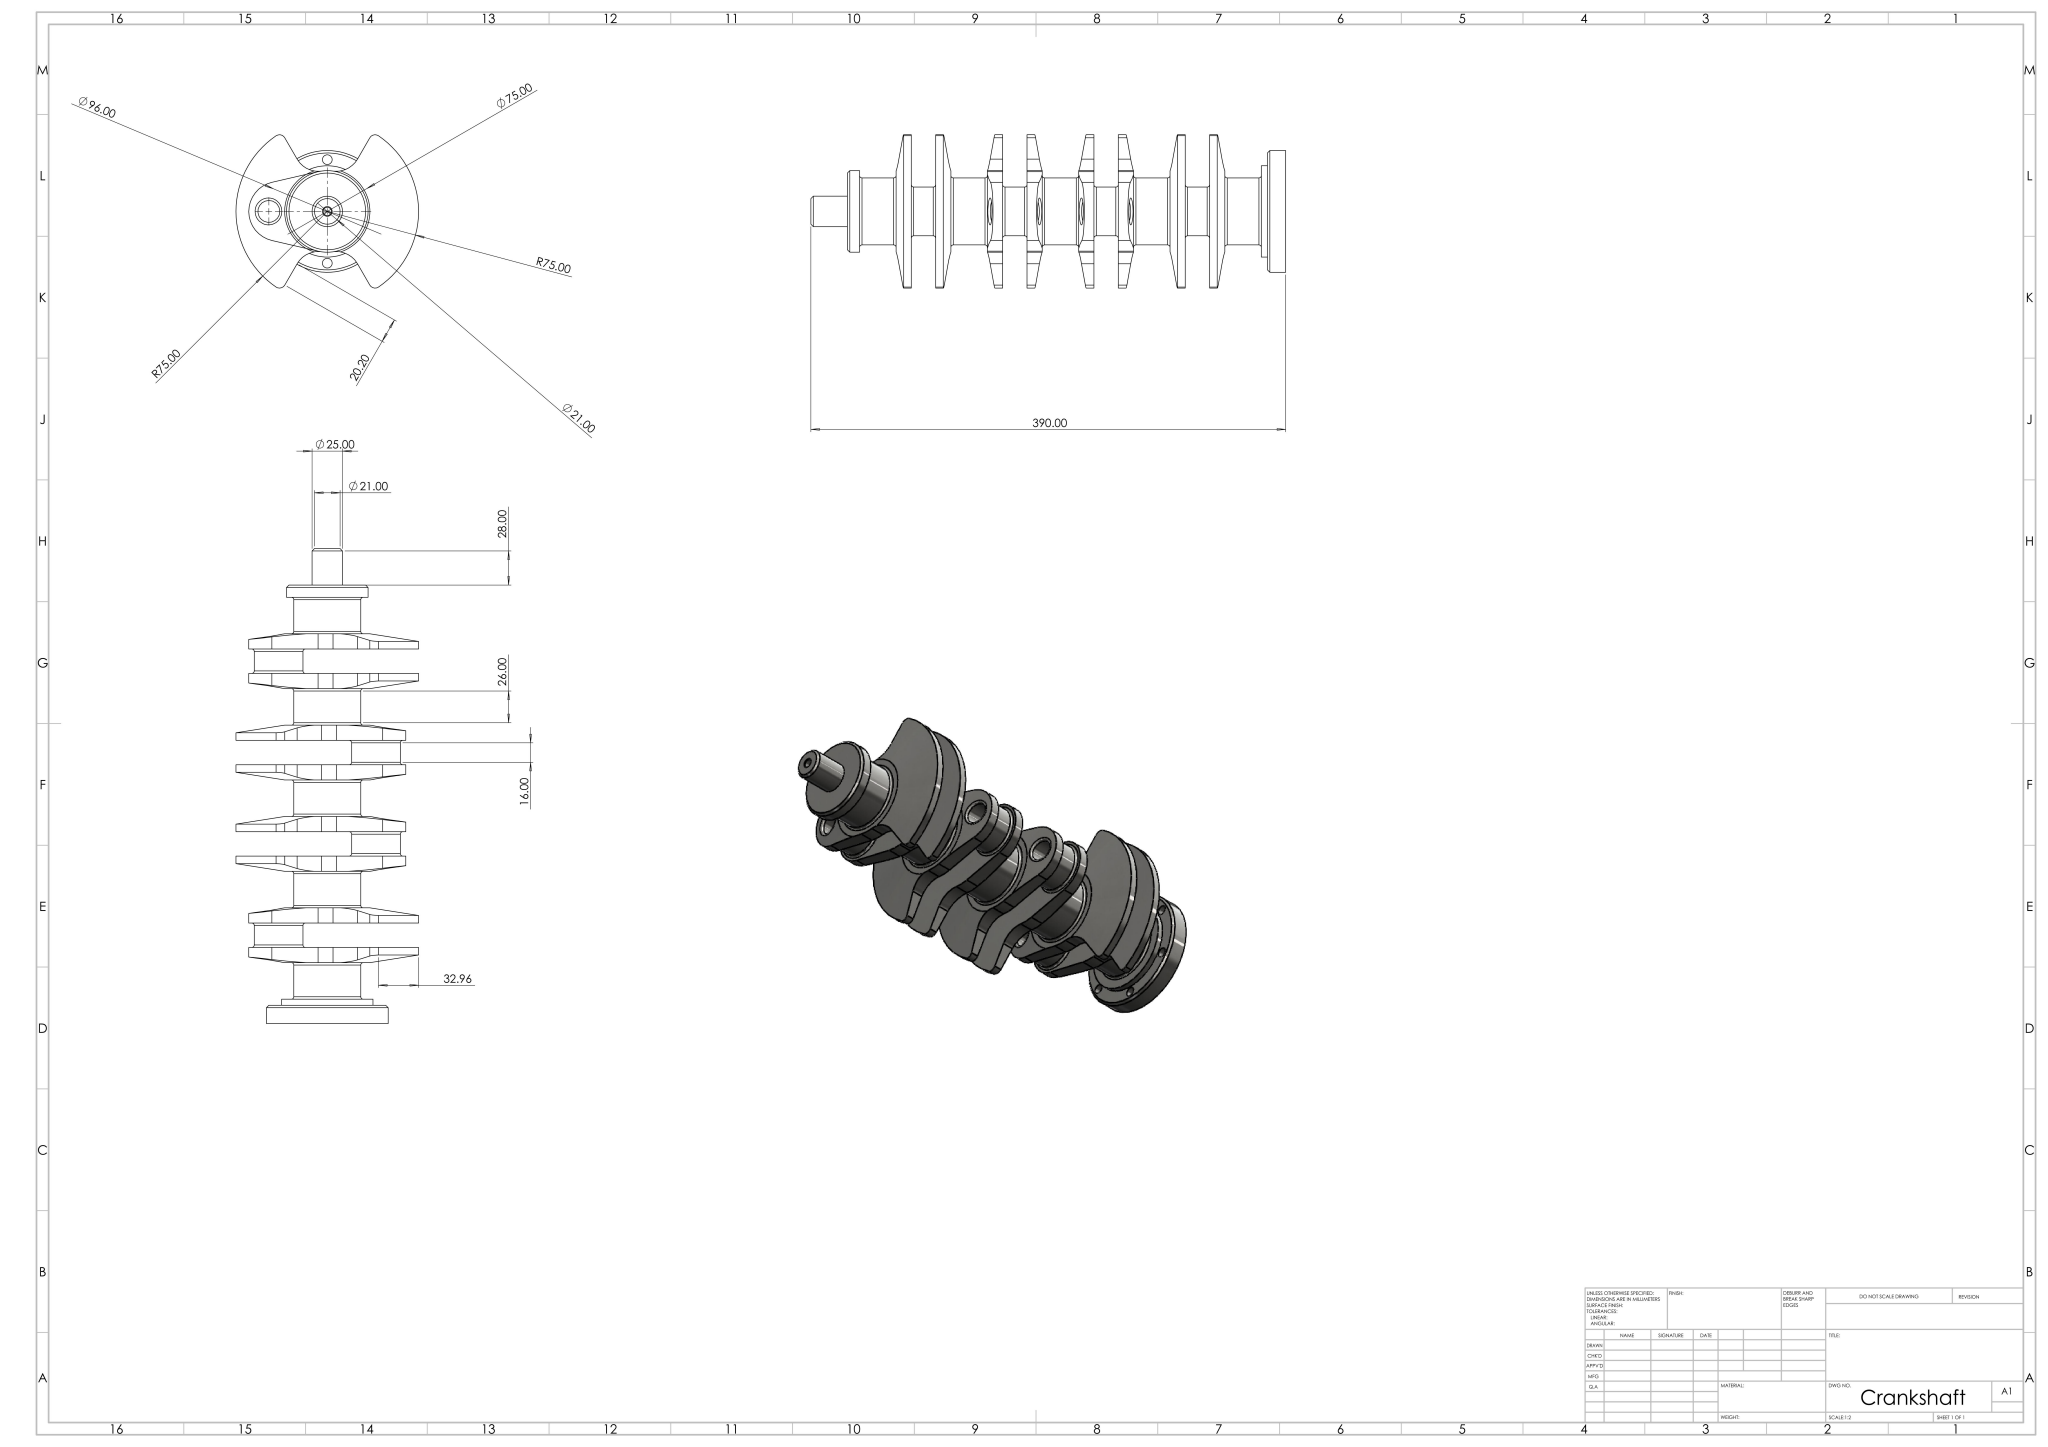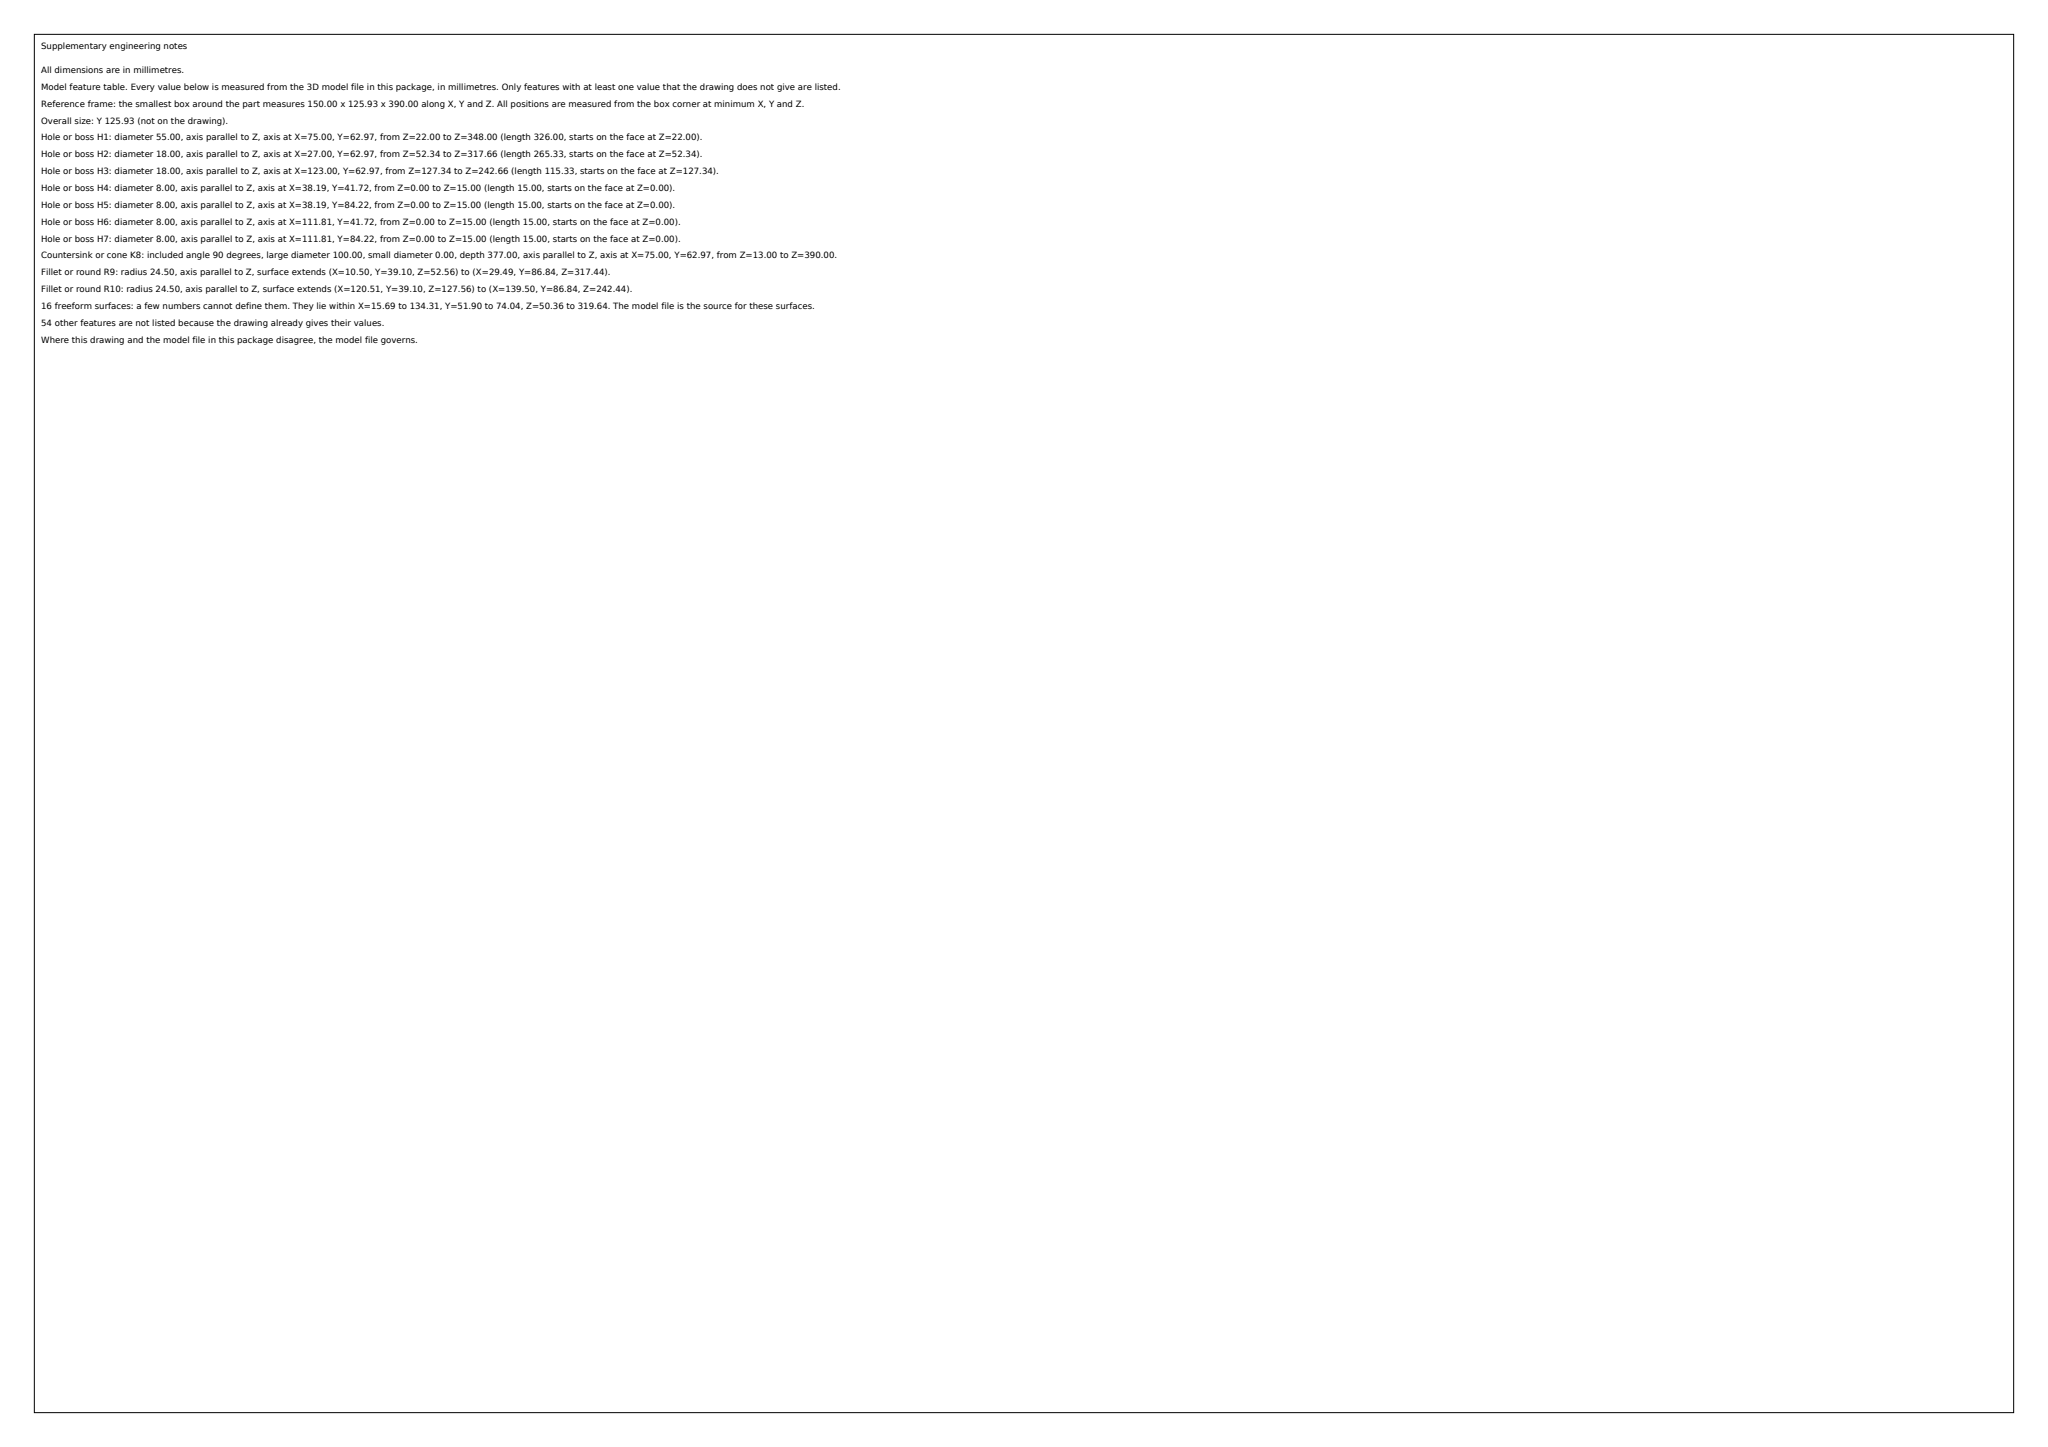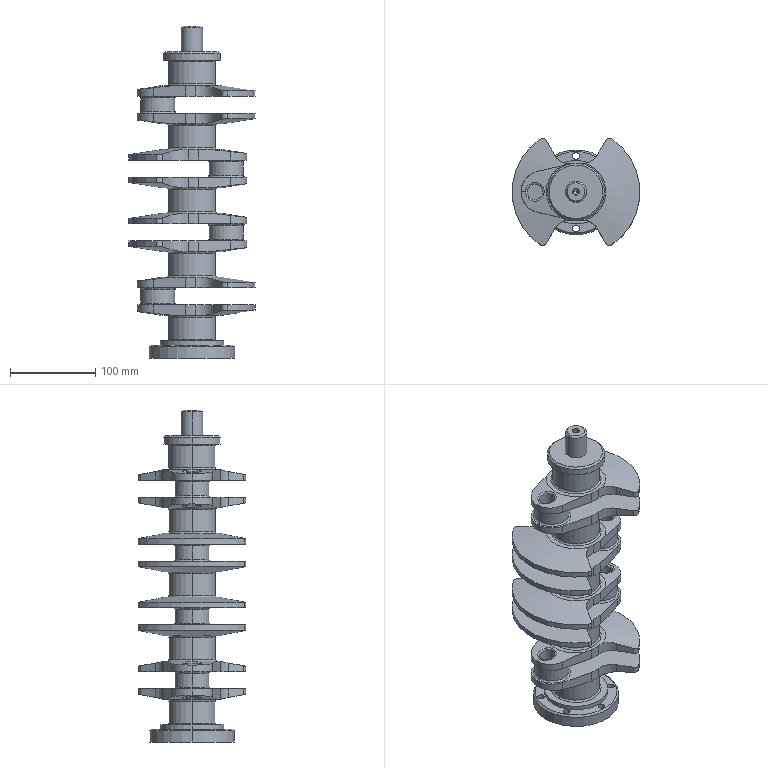Part | SolidWorks | mm | 1 solid | 260 faces | box 150 x 125.93 x 390 mm | volume 1436859 mm3 | cylinder 120 | plane 54 | torus 36 | cone 34 | spline 16 | commonest cylinder face diameters 40 x24 67 x18 49 x16 10 x16 8 x12 55 x10 18 x8 150 x8